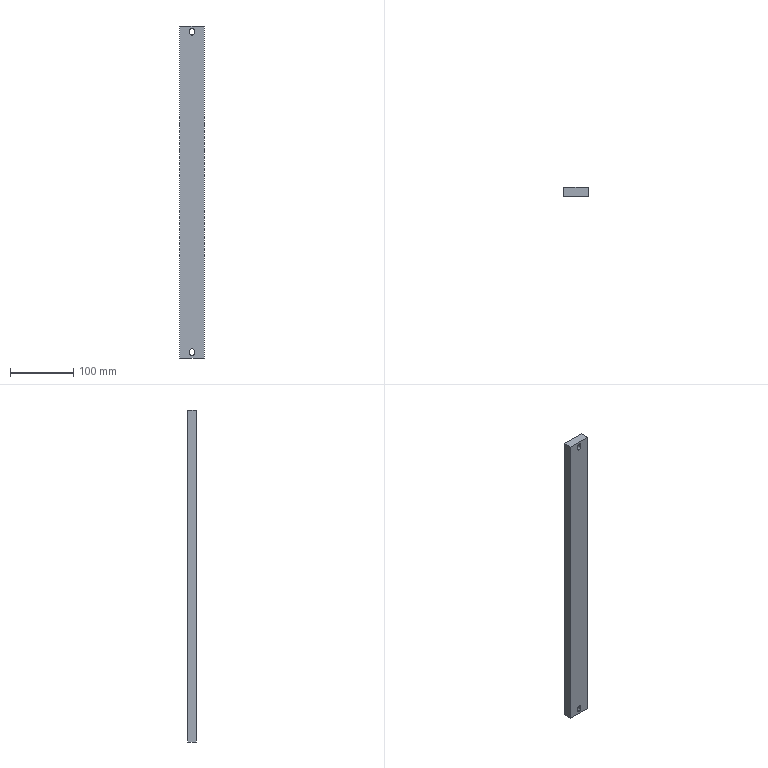Component | SolidWorks | CodingMachineSupport-1 | 1 solid | 16 faces | box 38 x 14 x 523 mm | volume 276374 mm3 | plane 10 | cylinder 6 | commonest cylinder face diameters 7 x6
build123d program:
from build123d import *

# Parameters (mm, degrees)
SKETCH1_W           = 523
SKETCH1_H           = 38
BOSS_EXTRUDE1_DEPTH = 14


with BuildPart() as part:
    # Sketch1 → Boss-Extrude1 (new body)
    with BuildSketch(Plane.XY.offset(7)):
        Rectangle(SKETCH1_W, SKETCH1_H)
        with BuildLine():
            Line((-250.5, -3.5), (-254.5, -3.5))
            ThreePointArc((-254.5, -3.5), (-258, 0), (-254.5, 3.5))
            Line((-254.5, 3.5), (-250.5, 3.5))
            ThreePointArc((-250.5, 3.5), (-247, 0), (-250.5, -3.5))
        make_face(mode=Mode.SUBTRACT)
        with BuildLine():
            Line((254.5, -3.5), (250.5, -3.5))
            ThreePointArc((250.5, -3.5), (247, 0), (250.5, 3.5))
            Line((250.5, 3.5), (254.5, 3.5))
            ThreePointArc((254.5, 3.5), (258, 0), (254.5, -3.5))
        make_face(mode=Mode.SUBTRACT)
    extrude(amount=-BOSS_EXTRUDE1_DEPTH)


solid = part.part

# Placed as in the assembly
solid = solid.moved(Location((-277, 365, 0), (90, 0, 90)))
STEP:
#1=CARTESIAN_POINT('',(-10.906,14.646,-10.157));
#2=VERTEX_POINT('',#1);
#3=CARTESIAN_POINT('',(-10.768,14.646,-10.02));
#4=VERTEX_POINT('',#3);
#5=CARTESIAN_POINT('',(-10.906,14.646,-10.02));
#6=DIRECTION('',(-0.,-1.,0.));
#7=DIRECTION('',(0.,0.,1.));
#8=AXIS2_PLACEMENT_3D('',#5,#6,#7);
#9=CIRCLE('',#8,0.1378);
#10=EDGE_CURVE('',#2,#4,#9,.T.);
#11=ORIENTED_EDGE('',*,*,#10,.F.);
#12=CARTESIAN_POINT('',(-10.906,14.094,-10.157));
#13=VERTEX_POINT('',#12);
#14=CARTESIAN_POINT('',(-10.906,14.646,-10.157));
#15=DIRECTION('',(-0.,-1.,0.));
#16=VECTOR('',#15,39.37);
#17=LINE('',#14,#16);
#18=EDGE_CURVE('',#2,#13,#17,.T.);
#19=ORIENTED_EDGE('',*,*,#18,.T.);
#20=CARTESIAN_POINT('',(-10.768,14.094,-10.02));
#21=VERTEX_POINT('',#20);
#22=CARTESIAN_POINT('',(-10.906,14.094,-10.02));
#23=DIRECTION('',(-0.,-1.,0.));
#24=DIRECTION('',(0.,0.,1.));
#25=AXIS2_PLACEMENT_3D('',#22,#23,#24);
#26=CIRCLE('',#25,0.1378);
#27=EDGE_CURVE('',#13,#21,#26,.T.);
#28=ORIENTED_EDGE('',*,*,#27,.T.);
#29=CARTESIAN_POINT('',(-10.768,14.646,-10.02));
#30=DIRECTION('',(-0.,-1.,0.));
#31=VECTOR('',#30,39.37);
#32=LINE('',#29,#31);
#33=EDGE_CURVE('',#4,#21,#32,.T.);
#34=ORIENTED_EDGE('',*,*,#33,.F.);
#35=EDGE_LOOP('',(#11,#19,#28,#34));
#36=FACE_OUTER_BOUND('',#35,.T.);
#37=CARTESIAN_POINT('',(-10.906,14.646,-10.02));
#38=DIRECTION('',(-0.,-1.,0.));
#39=DIRECTION('',(0.,0.,-1.));
#40=AXIS2_PLACEMENT_3D('',#37,#38,#39);
#41=CYLINDRICAL_SURFACE('',#40,0.1378);
#42=ADVANCED_FACE('',(#36),#41,.F.);
#43=CARTESIAN_POINT('',(-10.906,14.646,9.724));
#44=VERTEX_POINT('',#43);
#45=CARTESIAN_POINT('',(-10.768,14.646,9.862));
#46=VERTEX_POINT('',#45);
#47=CARTESIAN_POINT('',(-10.906,14.646,9.862));
#48=DIRECTION('',(-0.,-1.,0.));
#49=DIRECTION('',(0.,0.,1.));
#50=AXIS2_PLACEMENT_3D('',#47,#48,#49);
#51=CIRCLE('',#50,0.1378);
#52=EDGE_CURVE('',#44,#46,#51,.T.);
#53=ORIENTED_EDGE('',*,*,#52,.F.);
#54=CARTESIAN_POINT('',(-10.906,14.094,9.724));
#55=VERTEX_POINT('',#54);
#56=CARTESIAN_POINT('',(-10.906,14.646,9.724));
#57=DIRECTION('',(-0.,-1.,0.));
#58=VECTOR('',#57,39.37);
#59=LINE('',#56,#58);
#60=EDGE_CURVE('',#44,#55,#59,.T.);
#61=ORIENTED_EDGE('',*,*,#60,.T.);
#62=CARTESIAN_POINT('',(-10.768,14.094,9.862));
#63=VERTEX_POINT('',#62);
#64=CARTESIAN_POINT('',(-10.906,14.094,9.862));
#65=DIRECTION('',(-0.,-1.,0.));
#66=DIRECTION('',(0.,0.,1.));
#67=AXIS2_PLACEMENT_3D('',#64,#65,#66);
#68=CIRCLE('',#67,0.1378);
#69=EDGE_CURVE('',#55,#63,#68,.T.);
#70=ORIENTED_EDGE('',*,*,#69,.T.);
#71=CARTESIAN_POINT('',(-10.768,14.646,9.862));
#72=DIRECTION('',(-0.,-1.,0.));
#73=VECTOR('',#72,39.37);
#74=LINE('',#71,#73);
#75=EDGE_CURVE('',#46,#63,#74,.T.);
#76=ORIENTED_EDGE('',*,*,#75,.F.);
#77=EDGE_LOOP('',(#53,#61,#70,#76));
#78=FACE_OUTER_BOUND('',#77,.T.);
#79=CARTESIAN_POINT('',(-10.906,14.646,9.862));
#80=DIRECTION('',(-0.,-1.,0.));
#81=DIRECTION('',(0.,0.,-1.));
#82=AXIS2_PLACEMENT_3D('',#79,#80,#81);
#83=CYLINDRICAL_SURFACE('',#82,0.1378);
#84=ADVANCED_FACE('',(#78),#83,.F.);
#85=CARTESIAN_POINT('',(-11.654,14.094,10.295));
#86=VERTEX_POINT('',#85);
#87=CARTESIAN_POINT('',(-11.654,14.094,-10.295));
#88=VERTEX_POINT('',#87);
#89=CARTESIAN_POINT('',(-11.654,14.094,10.295));
#90=DIRECTION('',(-0.,-0.,-1.));
#91=VECTOR('',#90,39.37);
#92=LINE('',#89,#91);
#93=EDGE_CURVE('',#86,#88,#92,.T.);
#94=ORIENTED_EDGE('',*,*,#93,.F.);
#95=CARTESIAN_POINT('',(-11.654,14.646,10.295));
#96=VERTEX_POINT('',#95);
#97=CARTESIAN_POINT('',(-11.654,14.646,10.295));
#98=DIRECTION('',(-0.,-1.,0.));
#99=VECTOR('',#98,39.37);
#100=LINE('',#97,#99);
#101=EDGE_CURVE('',#96,#86,#100,.T.);
#102=ORIENTED_EDGE('',*,*,#101,.F.);
#103=CARTESIAN_POINT('',(-11.654,14.646,-10.295));
#104=VERTEX_POINT('',#103);
#105=CARTESIAN_POINT('',(-11.654,14.646,10.295));
#106=DIRECTION('',(-0.,-0.,-1.));
#107=VECTOR('',#106,39.37);
#108=LINE('',#105,#107);
#109=EDGE_CURVE('',#96,#104,#108,.T.);
#110=ORIENTED_EDGE('',*,*,#109,.T.);
#111=CARTESIAN_POINT('',(-11.654,14.646,-10.295));
#112=DIRECTION('',(-0.,-1.,0.));
#113=VECTOR('',#112,39.37);
#114=LINE('',#111,#113);
#115=EDGE_CURVE('',#104,#88,#114,.T.);
#116=ORIENTED_EDGE('',*,*,#115,.T.);
#117=EDGE_LOOP('',(#94,#102,#110,#116));
#118=FACE_OUTER_BOUND('',#117,.T.);
#119=CARTESIAN_POINT('',(-11.654,14.646,10.295));
#120=DIRECTION('',(-1.,0.,0.));
#121=DIRECTION('',(0.,1.,-0.));
#122=AXIS2_PLACEMENT_3D('',#119,#120,#121);
#123=PLANE('',#122);
#124=ADVANCED_FACE('',(#118),#123,.T.);
#125=CARTESIAN_POINT('',(-10.157,14.094,10.295));
#126=VERTEX_POINT('',#125);
#127=CARTESIAN_POINT('',(-10.157,14.094,10.295));
#128=DIRECTION('',(-1.,0.,0.));
#129=VECTOR('',#128,39.37);
#130=LINE('',#127,#129);
#131=EDGE_CURVE('',#126,#86,#130,.T.);
#132=ORIENTED_EDGE('',*,*,#131,.F.);
#133=CARTESIAN_POINT('',(-10.157,14.646,10.295));
#134=VERTEX_POINT('',#133);
#135=CARTESIAN_POINT('',(-10.157,14.646,10.295));
#136=DIRECTION('',(-0.,-1.,0.));
#137=VECTOR('',#136,39.37);
#138=LINE('',#135,#137);
#139=EDGE_CURVE('',#134,#126,#138,.T.);
#140=ORIENTED_EDGE('',*,*,#139,.F.);
#141=CARTESIAN_POINT('',(-10.157,14.646,10.295));
#142=DIRECTION('',(-1.,0.,0.));
#143=VECTOR('',#142,39.37);
#144=LINE('',#141,#143);
#145=EDGE_CURVE('',#134,#96,#144,.T.);
#146=ORIENTED_EDGE('',*,*,#145,.T.);
#147=ORIENTED_EDGE('',*,*,#101,.T.);
#148=EDGE_LOOP('',(#132,#140,#146,#147));
#149=FACE_OUTER_BOUND('',#148,.T.);
#150=CARTESIAN_POINT('',(-10.157,14.646,10.295));
#151=DIRECTION('',(0.,0.,1.));
#152=DIRECTION('',(-0.,-1.,0.));
#153=AXIS2_PLACEMENT_3D('',#150,#151,#152);
#154=PLANE('',#153);
#155=ADVANCED_FACE('',(#149),#154,.T.);
#156=CARTESIAN_POINT('',(-10.157,14.094,-10.295));
#157=VERTEX_POINT('',#156);
#158=CARTESIAN_POINT('',(-10.157,14.094,-10.295));
#159=DIRECTION('',(0.,0.,1.));
#160=VECTOR('',#159,39.37);
#161=LINE('',#158,#160);
#162=EDGE_CURVE('',#157,#126,#161,.T.);
#163=ORIENTED_EDGE('',*,*,#162,.F.);
#164=CARTESIAN_POINT('',(-10.157,14.646,-10.295));
#165=VERTEX_POINT('',#164);
#166=CARTESIAN_POINT('',(-10.157,14.646,-10.295));
#167=DIRECTION('',(-0.,-1.,0.));
#168=VECTOR('',#167,39.37);
#169=LINE('',#166,#168);
#170=EDGE_CURVE('',#165,#157,#169,.T.);
#171=ORIENTED_EDGE('',*,*,#170,.F.);
#172=CARTESIAN_POINT('',(-10.157,14.646,-10.295));
#173=DIRECTION('',(0.,0.,1.));
#174=VECTOR('',#173,39.37);
#175=LINE('',#172,#174);
#176=EDGE_CURVE('',#165,#134,#175,.T.);
#177=ORIENTED_EDGE('',*,*,#176,.T.);
#178=ORIENTED_EDGE('',*,*,#139,.T.);
#179=EDGE_LOOP('',(#163,#171,#177,#178));
#180=FACE_OUTER_BOUND('',#179,.T.);
#181=CARTESIAN_POINT('',(-10.157,14.646,-10.295));
#182=DIRECTION('',(1.,-0.,-0.));
#183=DIRECTION('',(0.,0.,1.));
#184=AXIS2_PLACEMENT_3D('',#181,#182,#183);
#185=PLANE('',#184);
#186=ADVANCED_FACE('',(#180),#185,.T.);
#187=CARTESIAN_POINT('',(-11.654,14.094,-10.295));
#188=DIRECTION('',(1.,-0.,-0.));
#189=VECTOR('',#188,39.37);
#190=LINE('',#187,#189);
#191=EDGE_CURVE('',#88,#157,#190,.T.);
#192=ORIENTED_EDGE('',*,*,#191,.F.);
#193=ORIENTED_EDGE('',*,*,#115,.F.);
#194=CARTESIAN_POINT('',(-11.654,14.646,-10.295));
#195=DIRECTION('',(1.,-0.,-0.));
#196=VECTOR('',#195,39.37);
#197=LINE('',#194,#196);
#198=EDGE_CURVE('',#104,#165,#197,.T.);
#199=ORIENTED_EDGE('',*,*,#198,.T.);
#200=ORIENTED_EDGE('',*,*,#170,.T.);
#201=EDGE_LOOP('',(#192,#193,#199,#200));
#202=FACE_OUTER_BOUND('',#201,.T.);
#203=CARTESIAN_POINT('',(-11.654,14.646,-10.295));
#204=DIRECTION('',(-0.,-0.,-1.));
#205=DIRECTION('',(0.,1.,-0.));
#206=AXIS2_PLACEMENT_3D('',#203,#204,#205);
#207=PLANE('',#206);
#208=ADVANCED_FACE('',(#202),#207,.T.);
#209=CARTESIAN_POINT('',(-11.043,14.646,-9.862));
#210=VERTEX_POINT('',#209);
#211=CARTESIAN_POINT('',(-11.043,14.646,-10.02));
#212=VERTEX_POINT('',#211);
#213=CARTESIAN_POINT('',(-11.043,14.646,-10.02));
#214=DIRECTION('',(0.,-0.,-1.));
#215=VECTOR('',#214,39.37);
#216=LINE('',#213,#215);
#217=EDGE_CURVE('',#210,#212,#216,.T.);
#218=ORIENTED_EDGE('',*,*,#217,.T.);
#219=CARTESIAN_POINT('',(-10.906,14.646,-10.02));
#220=DIRECTION('',(-0.,-1.,0.));
#221=DIRECTION('',(0.,0.,1.));
#222=AXIS2_PLACEMENT_3D('',#219,#220,#221);
#223=CIRCLE('',#222,0.1378);
#224=EDGE_CURVE('',#212,#2,#223,.T.);
#225=ORIENTED_EDGE('',*,*,#224,.T.);
#226=ORIENTED_EDGE('',*,*,#10,.T.);
#227=CARTESIAN_POINT('',(-10.768,14.646,-9.862));
#228=VERTEX_POINT('',#227);
#229=CARTESIAN_POINT('',(-10.768,14.646,-9.862));
#230=DIRECTION('',(0.,0.,1.));
#231=VECTOR('',#230,39.37);
#232=LINE('',#229,#231);
#233=EDGE_CURVE('',#4,#228,#232,.T.);
#234=ORIENTED_EDGE('',*,*,#233,.T.);
#235=CARTESIAN_POINT('',(-10.906,14.646,-9.862));
#236=DIRECTION('',(-0.,-1.,0.));
#237=DIRECTION('',(0.,0.,1.));
#238=AXIS2_PLACEMENT_3D('',#235,#236,#237);
#239=CIRCLE('',#238,0.1378);
#240=EDGE_CURVE('',#228,#210,#239,.T.);
#241=ORIENTED_EDGE('',*,*,#240,.T.);
#242=EDGE_LOOP('',(#218,#225,#226,#234,#241));
#243=FACE_BOUND('',#242,.T.);
#244=CARTESIAN_POINT('',(-11.043,14.646,10.02));
#245=VERTEX_POINT('',#244);
#246=CARTESIAN_POINT('',(-11.043,14.646,9.862));
#247=VERTEX_POINT('',#246);
#248=CARTESIAN_POINT('',(-11.043,14.646,9.862));
#249=DIRECTION('',(-0.,-0.,-1.));
#250=VECTOR('',#249,39.37);
#251=LINE('',#248,#250);
#252=EDGE_CURVE('',#245,#247,#251,.T.);
#253=ORIENTED_EDGE('',*,*,#252,.T.);
#254=CARTESIAN_POINT('',(-10.906,14.646,9.862));
#255=DIRECTION('',(-0.,-1.,0.));
#256=DIRECTION('',(0.,0.,1.));
#257=AXIS2_PLACEMENT_3D('',#254,#255,#256);
#258=CIRCLE('',#257,0.1378);
#259=EDGE_CURVE('',#247,#44,#258,.T.);
#260=ORIENTED_EDGE('',*,*,#259,.T.);
#261=ORIENTED_EDGE('',*,*,#52,.T.);
#262=CARTESIAN_POINT('',(-10.768,14.646,10.02));
#263=VERTEX_POINT('',#262);
#264=CARTESIAN_POINT('',(-10.768,14.646,10.02));
#265=DIRECTION('',(0.,0.,1.));
#266=VECTOR('',#265,39.37);
#267=LINE('',#264,#266);
#268=EDGE_CURVE('',#46,#263,#267,.T.);
#269=ORIENTED_EDGE('',*,*,#268,.T.);
#270=CARTESIAN_POINT('',(-10.906,14.646,10.02));
#271=DIRECTION('',(-0.,-1.,0.));
#272=DIRECTION('',(0.,0.,1.));
#273=AXIS2_PLACEMENT_3D('',#270,#271,#272);
#274=CIRCLE('',#273,0.1378);
#275=EDGE_CURVE('',#263,#245,#274,.T.);
#276=ORIENTED_EDGE('',*,*,#275,.T.);
#277=EDGE_LOOP('',(#253,#260,#261,#269,#276));
#278=FACE_BOUND('',#277,.T.);
#279=ORIENTED_EDGE('',*,*,#109,.F.);
#280=ORIENTED_EDGE('',*,*,#145,.F.);
#281=ORIENTED_EDGE('',*,*,#176,.F.);
#282=ORIENTED_EDGE('',*,*,#198,.F.);
#283=EDGE_LOOP('',(#279,#280,#281,#282));
#284=FACE_OUTER_BOUND('',#283,.T.);
#285=CARTESIAN_POINT('',(-10.906,14.646,-0.));
#286=DIRECTION('',(-0.,-1.,0.));
#287=DIRECTION('',(-0.,-0.,-1.));
#288=AXIS2_PLACEMENT_3D('',#285,#286,#287);
#289=PLANE('',#288);
#290=ADVANCED_FACE('',(#243,#278,#284),#289,.F.);
#291=CARTESIAN_POINT('',(-11.043,14.094,-10.02));
#292=VERTEX_POINT('',#291);
#293=CARTESIAN_POINT('',(-10.906,14.094,-10.02));
#294=DIRECTION('',(-0.,-1.,0.));
#295=DIRECTION('',(0.,0.,1.));
#296=AXIS2_PLACEMENT_3D('',#293,#294,#295);
#297=CIRCLE('',#296,0.1378);
#298=EDGE_CURVE('',#292,#13,#297,.T.);
#299=ORIENTED_EDGE('',*,*,#298,.F.);
#300=CARTESIAN_POINT('',(-11.043,14.094,-9.862));
#301=VERTEX_POINT('',#300);
#302=CARTESIAN_POINT('',(-11.043,14.094,-10.02));
#303=DIRECTION('',(0.,-0.,-1.));
#304=VECTOR('',#303,39.37);
#305=LINE('',#302,#304);
#306=EDGE_CURVE('',#301,#292,#305,.T.);
#307=ORIENTED_EDGE('',*,*,#306,.F.);
#308=CARTESIAN_POINT('',(-10.768,14.094,-9.862));
#309=VERTEX_POINT('',#308);
#310=CARTESIAN_POINT('',(-10.906,14.094,-9.862));
#311=DIRECTION('',(-0.,-1.,0.));
#312=DIRECTION('',(0.,0.,1.));
#313=AXIS2_PLACEMENT_3D('',#310,#311,#312);
#314=CIRCLE('',#313,0.1378);
#315=EDGE_CURVE('',#309,#301,#314,.T.);
#316=ORIENTED_EDGE('',*,*,#315,.F.);
#317=CARTESIAN_POINT('',(-10.768,14.094,-9.862));
#318=DIRECTION('',(0.,0.,1.));
#319=VECTOR('',#318,39.37);
#320=LINE('',#317,#319);
#321=EDGE_CURVE('',#21,#309,#320,.T.);
#322=ORIENTED_EDGE('',*,*,#321,.F.);
#323=ORIENTED_EDGE('',*,*,#27,.F.);
#324=EDGE_LOOP('',(#299,#307,#316,#322,#323));
#325=FACE_BOUND('',#324,.T.);
#326=CARTESIAN_POINT('',(-11.043,14.094,9.862));
#327=VERTEX_POINT('',#326);
#328=CARTESIAN_POINT('',(-10.906,14.094,9.862));
#329=DIRECTION('',(-0.,-1.,0.));
#330=DIRECTION('',(0.,0.,1.));
#331=AXIS2_PLACEMENT_3D('',#328,#329,#330);
#332=CIRCLE('',#331,0.1378);
#333=EDGE_CURVE('',#327,#55,#332,.T.);
#334=ORIENTED_EDGE('',*,*,#333,.F.);
#335=CARTESIAN_POINT('',(-11.043,14.094,10.02));
#336=VERTEX_POINT('',#335);
#337=CARTESIAN_POINT('',(-11.043,14.094,9.862));
#338=DIRECTION('',(-0.,-0.,-1.));
#339=VECTOR('',#338,39.37);
#340=LINE('',#337,#339);
#341=EDGE_CURVE('',#336,#327,#340,.T.);
#342=ORIENTED_EDGE('',*,*,#341,.F.);
#343=CARTESIAN_POINT('',(-10.768,14.094,10.02));
#344=VERTEX_POINT('',#343);
#345=CARTESIAN_POINT('',(-10.906,14.094,10.02));
#346=DIRECTION('',(-0.,-1.,0.));
#347=DIRECTION('',(0.,0.,1.));
#348=AXIS2_PLACEMENT_3D('',#345,#346,#347);
#349=CIRCLE('',#348,0.1378);
#350=EDGE_CURVE('',#344,#336,#349,.T.);
#351=ORIENTED_EDGE('',*,*,#350,.F.);
#352=CARTESIAN_POINT('',(-10.768,14.094,10.02));
#353=DIRECTION('',(0.,0.,1.));
#354=VECTOR('',#353,39.37);
#355=LINE('',#352,#354);
#356=EDGE_CURVE('',#63,#344,#355,.T.);
#357=ORIENTED_EDGE('',*,*,#356,.F.);
#358=ORIENTED_EDGE('',*,*,#69,.F.);
#359=EDGE_LOOP('',(#334,#342,#351,#357,#358));
#360=FACE_BOUND('',#359,.T.);
#361=ORIENTED_EDGE('',*,*,#93,.T.);
#362=ORIENTED_EDGE('',*,*,#191,.T.);
#363=ORIENTED_EDGE('',*,*,#162,.T.);
#364=ORIENTED_EDGE('',*,*,#131,.T.);
#365=EDGE_LOOP('',(#361,#362,#363,#364));
#366=FACE_OUTER_BOUND('',#365,.T.);
#367=CARTESIAN_POINT('',(-10.906,14.094,-0.));
#368=DIRECTION('',(-0.,-1.,0.));
#369=DIRECTION('',(-0.,-0.,-1.));
#370=AXIS2_PLACEMENT_3D('',#367,#368,#369);
#371=PLANE('',#370);
#372=ADVANCED_FACE('',(#325,#360,#366),#371,.T.);
#373=ORIENTED_EDGE('',*,*,#60,.F.);
#374=ORIENTED_EDGE('',*,*,#259,.F.);
#375=CARTESIAN_POINT('',(-11.043,14.646,9.862));
#376=DIRECTION('',(-0.,-1.,0.));
#377=VECTOR('',#376,39.37);
#378=LINE('',#375,#377);
#379=EDGE_CURVE('',#247,#327,#378,.T.);
#380=ORIENTED_EDGE('',*,*,#379,.T.);
#381=ORIENTED_EDGE('',*,*,#333,.T.);
#382=EDGE_LOOP('',(#373,#374,#380,#381));
#383=FACE_OUTER_BOUND('',#382,.T.);
#384=CARTESIAN_POINT('',(-10.906,14.646,9.862));
#385=DIRECTION('',(-0.,-1.,0.));
#386=DIRECTION('',(0.,0.,-1.));
#387=AXIS2_PLACEMENT_3D('',#384,#385,#386);
#388=CYLINDRICAL_SURFACE('',#387,0.1378);
#389=ADVANCED_FACE('',(#383),#388,.F.);
#390=ORIENTED_EDGE('',*,*,#341,.T.);
#391=ORIENTED_EDGE('',*,*,#379,.F.);
#392=ORIENTED_EDGE('',*,*,#252,.F.);
#393=CARTESIAN_POINT('',(-11.043,14.646,10.02));
#394=DIRECTION('',(-0.,-1.,0.));
#395=VECTOR('',#394,39.37);
#396=LINE('',#393,#395);
#397=EDGE_CURVE('',#245,#336,#396,.T.);
#398=ORIENTED_EDGE('',*,*,#397,.T.);
#399=EDGE_LOOP('',(#390,#391,#392,#398));
#400=FACE_OUTER_BOUND('',#399,.T.);
#401=CARTESIAN_POINT('',(-11.043,14.646,9.862));
#402=DIRECTION('',(-1.,0.,0.));
#403=DIRECTION('',(-0.,-0.,-1.));
#404=AXIS2_PLACEMENT_3D('',#401,#402,#403);
#405=PLANE('',#404);
#406=ADVANCED_FACE('',(#400),#405,.F.);
#407=ORIENTED_EDGE('',*,*,#350,.T.);
#408=ORIENTED_EDGE('',*,*,#397,.F.);
#409=ORIENTED_EDGE('',*,*,#275,.F.);
#410=CARTESIAN_POINT('',(-10.768,14.646,10.02));
#411=DIRECTION('',(-0.,-1.,0.));
#412=VECTOR('',#411,39.37);
#413=LINE('',#410,#412);
#414=EDGE_CURVE('',#263,#344,#413,.T.);
#415=ORIENTED_EDGE('',*,*,#414,.T.);
#416=EDGE_LOOP('',(#407,#408,#409,#415));
#417=FACE_OUTER_BOUND('',#416,.T.);
#418=CARTESIAN_POINT('',(-10.906,14.646,10.02));
#419=DIRECTION('',(-0.,-1.,0.));
#420=DIRECTION('',(0.,0.,-1.));
#421=AXIS2_PLACEMENT_3D('',#418,#419,#420);
#422=CYLINDRICAL_SURFACE('',#421,0.1378);
#423=ADVANCED_FACE('',(#417),#422,.F.);
#424=ORIENTED_EDGE('',*,*,#356,.T.);
#425=ORIENTED_EDGE('',*,*,#414,.F.);
#426=ORIENTED_EDGE('',*,*,#268,.F.);
#427=ORIENTED_EDGE('',*,*,#75,.T.);
#428=EDGE_LOOP('',(#424,#425,#426,#427));
#429=FACE_OUTER_BOUND('',#428,.T.);
#430=CARTESIAN_POINT('',(-10.768,14.646,10.02));
#431=DIRECTION('',(1.,-0.,-0.));
#432=DIRECTION('',(0.,0.,1.));
#433=AXIS2_PLACEMENT_3D('',#430,#431,#432);
#434=PLANE('',#433);
#435=ADVANCED_FACE('',(#429),#434,.F.);
#436=ORIENTED_EDGE('',*,*,#18,.F.);
#437=ORIENTED_EDGE('',*,*,#224,.F.);
#438=CARTESIAN_POINT('',(-11.043,14.646,-10.02));
#439=DIRECTION('',(-0.,-1.,0.));
#440=VECTOR('',#439,39.37);
#441=LINE('',#438,#440);
#442=EDGE_CURVE('',#212,#292,#441,.T.);
#443=ORIENTED_EDGE('',*,*,#442,.T.);
#444=ORIENTED_EDGE('',*,*,#298,.T.);
#445=EDGE_LOOP('',(#436,#437,#443,#444));
#446=FACE_OUTER_BOUND('',#445,.T.);
#447=CARTESIAN_POINT('',(-10.906,14.646,-10.02));
#448=DIRECTION('',(-0.,-1.,0.));
#449=DIRECTION('',(0.,0.,-1.));
#450=AXIS2_PLACEMENT_3D('',#447,#448,#449);
#451=CYLINDRICAL_SURFACE('',#450,0.1378);
#452=ADVANCED_FACE('',(#446),#451,.F.);
#453=ORIENTED_EDGE('',*,*,#306,.T.);
#454=ORIENTED_EDGE('',*,*,#442,.F.);
#455=ORIENTED_EDGE('',*,*,#217,.F.);
#456=CARTESIAN_POINT('',(-11.043,14.646,-9.862));
#457=DIRECTION('',(-0.,-1.,0.));
#458=VECTOR('',#457,39.37);
#459=LINE('',#456,#458);
#460=EDGE_CURVE('',#210,#301,#459,.T.);
#461=ORIENTED_EDGE('',*,*,#460,.T.);
#462=EDGE_LOOP('',(#453,#454,#455,#461));
#463=FACE_OUTER_BOUND('',#462,.T.);
#464=CARTESIAN_POINT('',(-11.043,14.646,-10.02));
#465=DIRECTION('',(-1.,0.,-0.));
#466=DIRECTION('',(0.,-0.,-1.));
#467=AXIS2_PLACEMENT_3D('',#464,#465,#466);
#468=PLANE('',#467);
#469=ADVANCED_FACE('',(#463),#468,.F.);
#470=ORIENTED_EDGE('',*,*,#315,.T.);
#471=ORIENTED_EDGE('',*,*,#460,.F.);
#472=ORIENTED_EDGE('',*,*,#240,.F.);
#473=CARTESIAN_POINT('',(-10.768,14.646,-9.862));
#474=DIRECTION('',(-0.,-1.,0.));
#475=VECTOR('',#474,39.37);
#476=LINE('',#473,#475);
#477=EDGE_CURVE('',#228,#309,#476,.T.);
#478=ORIENTED_EDGE('',*,*,#477,.T.);
#479=EDGE_LOOP('',(#470,#471,#472,#478));
#480=FACE_OUTER_BOUND('',#479,.T.);
#481=CARTESIAN_POINT('',(-10.906,14.646,-9.862));
#482=DIRECTION('',(-0.,-1.,0.));
#483=DIRECTION('',(0.,0.,-1.));
#484=AXIS2_PLACEMENT_3D('',#481,#482,#483);
#485=CYLINDRICAL_SURFACE('',#484,0.1378);
#486=ADVANCED_FACE('',(#480),#485,.F.);
#487=ORIENTED_EDGE('',*,*,#321,.T.);
#488=ORIENTED_EDGE('',*,*,#477,.F.);
#489=ORIENTED_EDGE('',*,*,#233,.F.);
#490=ORIENTED_EDGE('',*,*,#33,.T.);
#491=EDGE_LOOP('',(#487,#488,#489,#490));
#492=FACE_OUTER_BOUND('',#491,.T.);
#493=CARTESIAN_POINT('',(-10.768,14.646,-9.862));
#494=DIRECTION('',(1.,-0.,-0.));
#495=DIRECTION('',(0.,0.,1.));
#496=AXIS2_PLACEMENT_3D('',#493,#494,#495);
#497=PLANE('',#496);
#498=ADVANCED_FACE('',(#492),#497,.F.);
#499=CLOSED_SHELL('',(#42,#84,#124,#155,#186,#208,#290,#372,#389,#406,#423,#435,#452,#469,#486,#498));
#500=MANIFOLD_SOLID_BREP('',#499);
#501=CARTESIAN_POINT('',(0.,0.,0.));
#502=DIRECTION('',(0.,0.,1.));
#503=DIRECTION('',(1.,0.,0.));
#504=AXIS2_PLACEMENT_3D('',#501,#502,#503);
#505=(LENGTH_UNIT()NAMED_UNIT(*)SI_UNIT($,.METRE.));
#506=LENGTH_MEASURE_WITH_UNIT(LENGTH_MEASURE(0.0254),#505);
#507=DIMENSIONAL_EXPONENTS(1.,0.,0.,0.,0.,0.,0.);
#508=(CONVERSION_BASED_UNIT('',#506)LENGTH_UNIT()NAMED_UNIT(#507));
#509=UNCERTAINTY_MEASURE_WITH_UNIT(LENGTH_MEASURE(0.00001),#508,'','');
#510=(NAMED_UNIT(*)PLANE_ANGLE_UNIT()SI_UNIT($,.RADIAN.));
#511=(NAMED_UNIT(*)SI_UNIT($,.STERADIAN.)SOLID_ANGLE_UNIT());
#512=(GEOMETRIC_REPRESENTATION_CONTEXT(3)GLOBAL_UNCERTAINTY_ASSIGNED_CONTEXT((#509))GLOBAL_UNIT_ASSIGNED_CONTEXT((#508,#510,#511))REPRESENTATION_CONTEXT('',''));
#513=ADVANCED_BREP_SHAPE_REPRESENTATION('',(#500,#504),#512);
#514=COLOUR_RGB('',0.7922,0.8196,0.9333);
#515=FILL_AREA_STYLE_COLOUR('',#514);
#516=FILL_AREA_STYLE('',(#515));
#517=SURFACE_STYLE_FILL_AREA(#516);
#518=SURFACE_SIDE_STYLE('',(#517));
#519=SURFACE_STYLE_USAGE(.BOTH.,#518);
#520=PRESENTATION_STYLE_ASSIGNMENT((#519));
#521=STYLED_ITEM('',(#520),#500);
#522=PRESENTATION_LAYER_ASSIGNMENT('','',(#521));
#523=(LENGTH_UNIT()NAMED_UNIT(*)SI_UNIT($,.METRE.));
#524=LENGTH_MEASURE_WITH_UNIT(LENGTH_MEASURE(0.0254),#523);
#525=DIMENSIONAL_EXPONENTS(1.,0.,0.,0.,0.,0.,0.);
#526=(CONVERSION_BASED_UNIT('',#524)LENGTH_UNIT()NAMED_UNIT(#525));
#527=UNCERTAINTY_MEASURE_WITH_UNIT(LENGTH_MEASURE(0.00001),#526,'','');
#528=(NAMED_UNIT(*)PLANE_ANGLE_UNIT()SI_UNIT($,.RADIAN.));
#529=(NAMED_UNIT(*)SI_UNIT($,.STERADIAN.)SOLID_ANGLE_UNIT());
#530=(GEOMETRIC_REPRESENTATION_CONTEXT(3)GLOBAL_UNCERTAINTY_ASSIGNED_CONTEXT((#527))GLOBAL_UNIT_ASSIGNED_CONTEXT((#526,#528,#529))REPRESENTATION_CONTEXT('',''));
#531=MECHANICAL_DESIGN_GEOMETRIC_PRESENTATION_REPRESENTATION('',(#521),#530);